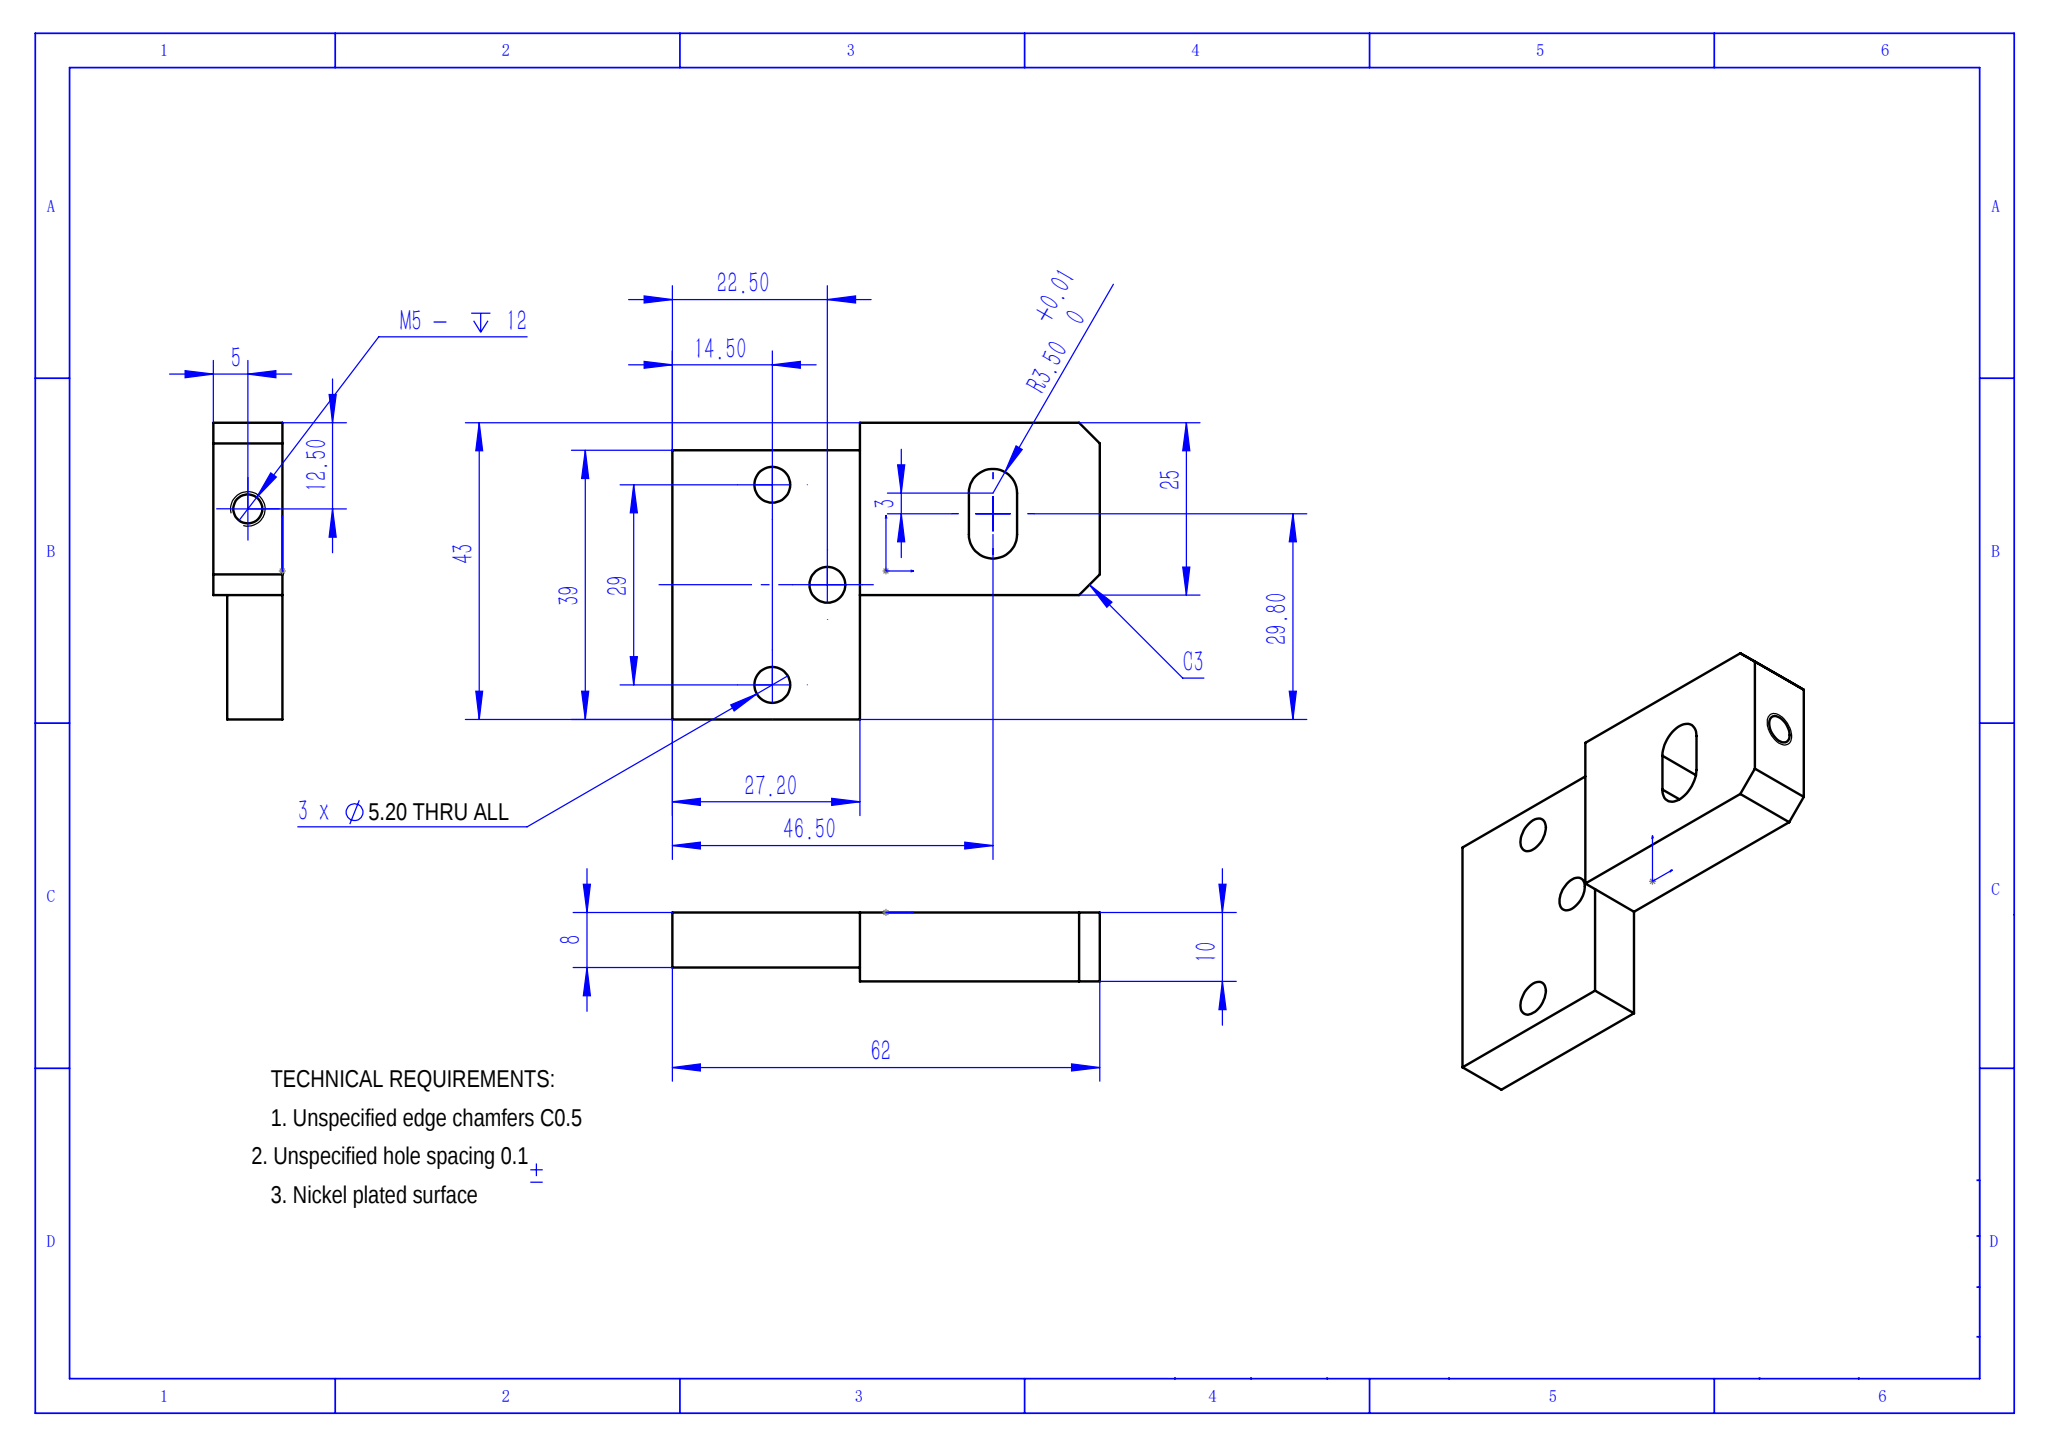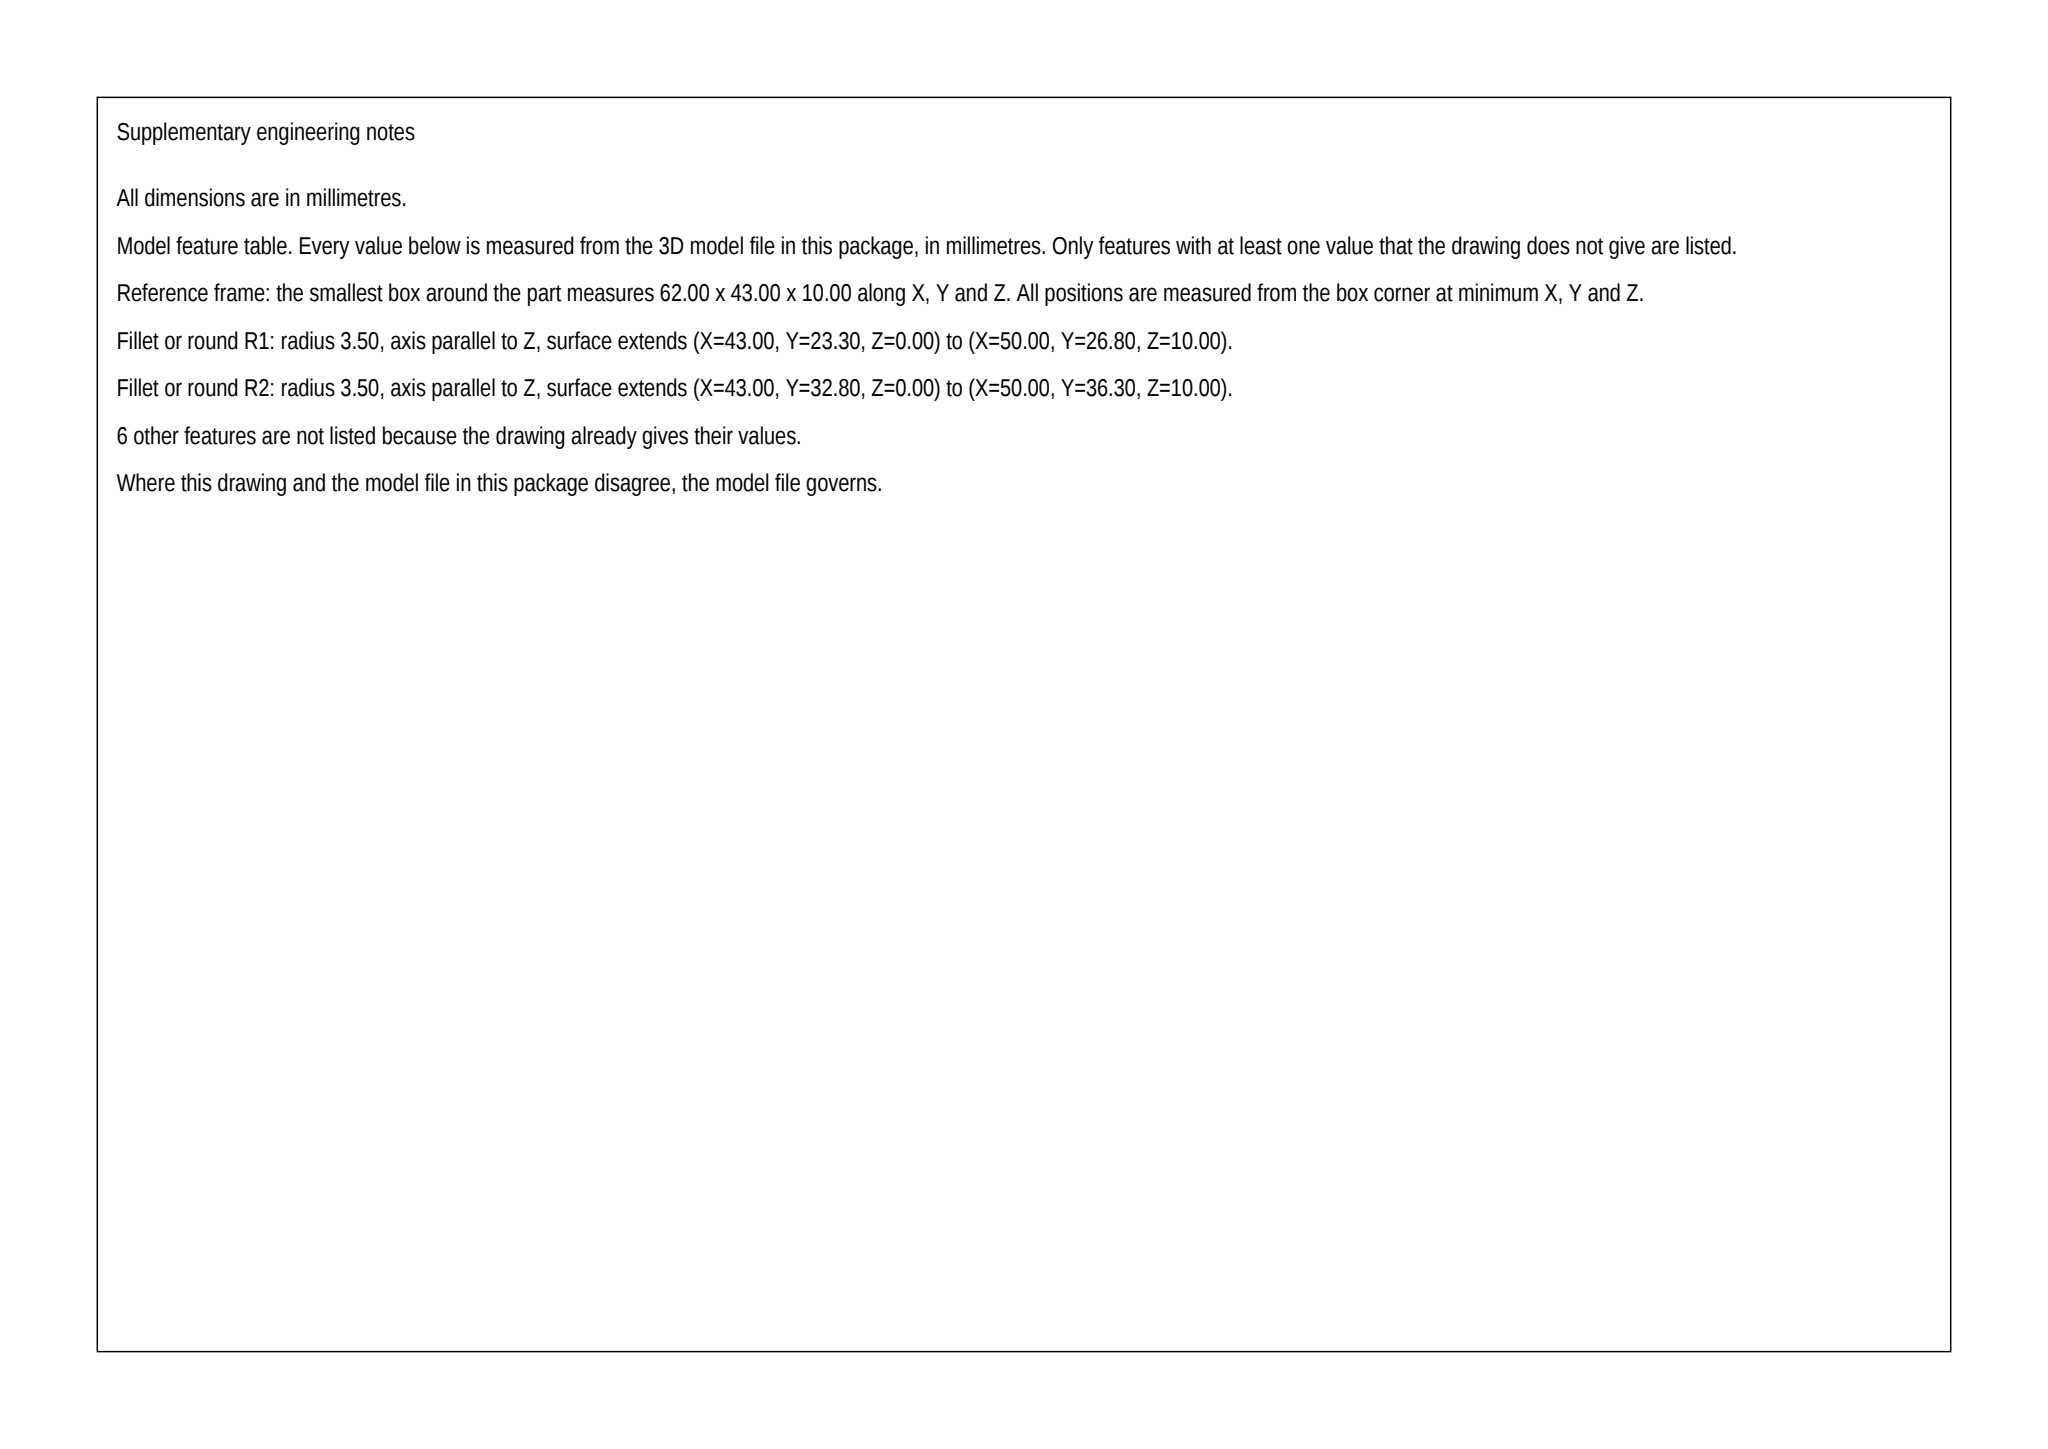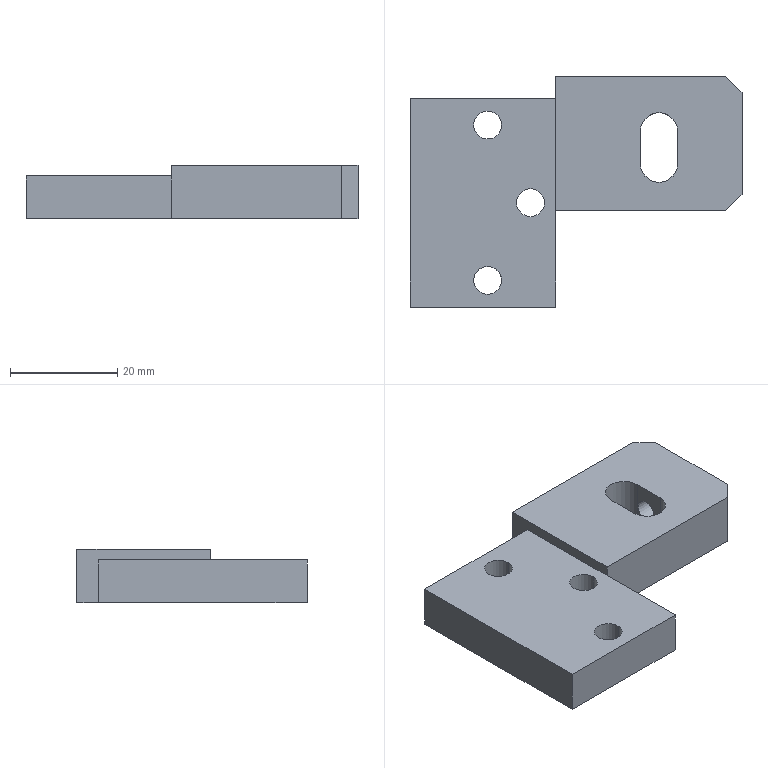Part | SolidWorks | mm | 1 solid | 25 faces | box 62 x 43 x 10 mm | volume 15616 mm3 | plane 15 | cylinder 10 | commonest cylinder face diameters 5.2 x6 4.2 x2 7 x2
build123d program:
from build123d import *

# Parameters (mm, degrees)
SKETCH1_W                  = 62
SKETCH1_H                  = 43
BOSS_EXTRUDE1_DEPTH        = 10
SKETCH2_W                  = 27.2
SKETCH2_H                  = 43
CUT_EXTRUDE1_DEPTH         = 2
SKETCH3_W                  = 27.2
SKETCH3_H                  = 4
CUT_EXTRUDE2_DEPTH         = 39.565
SKETCH7_W                  = 34.8
SKETCH7_H                  = 18
CUT_EXTRUDE3_DEPTH         = 40.029
F_5_2_5_2_DIAMETER_HOLE1_D = 5.2
CUT_EXTRUDE4_DEPTH         = 40.029
CHAMFER1_SIZE              = 3
M5_TAPPED_HOLE1_D          = 4.2
M5_TAPPED_HOLE1_DEPTH      = 14.4
M5_TAPPED_HOLE1_TIP        = 1.262


with BuildPart() as part:
    # Sketch1 → Boss-Extrude1 (new body)
    with BuildSketch(Plane.XY):
        Rectangle(SKETCH1_W, SKETCH1_H)
    extrude(amount=BOSS_EXTRUDE1_DEPTH)

    # Sketch2 → Cut-Extrude1 (cut)
    with BuildSketch(Plane.XY.offset(10)):
        with Locations((-17.4, 0)):
            Rectangle(SKETCH2_W, SKETCH2_H)
    extrude(amount=-CUT_EXTRUDE1_DEPTH, mode=Mode.SUBTRACT)

    # Sketch3 → Cut-Extrude2 (cut, through all)
    with BuildSketch(Plane.XY.offset(8)):
        with Locations((-17.4, 19.5)):
            Rectangle(SKETCH3_W, SKETCH3_H)
    extrude(amount=-CUT_EXTRUDE2_DEPTH, mode=Mode.SUBTRACT)

    # Sketch7 → Cut-Extrude3 (cut, through all)
    with BuildSketch(Plane.XY.offset(10)):
        with Locations((13.6, -12.5)):
            Rectangle(SKETCH7_W, SKETCH7_H)
    extrude(amount=-CUT_EXTRUDE3_DEPTH, mode=Mode.SUBTRACT)

    # 5.2 _5.2_ Diameter Hole1 (through all)
    with Locations(Plane(origin=(-16.5, 12.5, 0), x_dir=(-1, 0, 0), z_dir=(0, 0, -1))):
        with Locations((0, 0), (0, -29), (-8, -14.5)):
            Hole(F_5_2_5_2_DIAMETER_HOLE1_D / 2)

    # Sketch11 → Cut-Extrude4 (cut, through all)
    with BuildSketch(Plane.XY.offset(10)):
        with BuildLine():
            Line((12, 5.3), (12, 11.3))
            ThreePointArc((12, 11.3), (15.5, 14.8), (19, 11.3))
            Line((19, 11.3), (19, 5.3))
            ThreePointArc((19, 5.3), (15.5, 1.8), (12, 5.3))
        make_face()
    extrude(amount=-CUT_EXTRUDE4_DEPTH, mode=Mode.SUBTRACT)

    # Chamfer1
    chamfer1_edges = [part.edges().sort_by_distance(p)[0] for p in [
        (31, -3.5, 5),
        (31, 21.5, 5),
    ]]
    chamfer(chamfer1_edges, length=CHAMFER1_SIZE)

    # M5 Tapped Hole1
    with Locations(Plane(origin=(31, 9, 5), x_dir=(0, 1, 0), z_dir=(1, 0, 0))):
        with Locations((0, 0)):
            Hole(M5_TAPPED_HOLE1_D / 2, depth=M5_TAPPED_HOLE1_DEPTH)
            with Locations((0, 0, -(M5_TAPPED_HOLE1_DEPTH + M5_TAPPED_HOLE1_TIP / 2))):  # 118° drill point
                Cone(0, M5_TAPPED_HOLE1_D / 2, M5_TAPPED_HOLE1_TIP, mode=Mode.SUBTRACT)


solid = part.part
STEP:
#1=CARTESIAN_POINT('',(19.,9.,7.1));
#2=VERTEX_POINT('',#1);
#3=CARTESIAN_POINT('',(19.,9.,2.9));
#4=VERTEX_POINT('',#3);
#5=CARTESIAN_POINT('',(19.,9.,5.));
#6=DIRECTION('',(1.,0.,0.));
#7=DIRECTION('',(0.,0.,-1.));
#8=AXIS2_PLACEMENT_3D('',#5,#6,#7);
#9=CIRCLE('',#8,2.1);
#10=EDGE_CURVE('',#2,#4,#9,.T.);
#11=ORIENTED_EDGE('',*,*,#10,.F.);
#12=CARTESIAN_POINT('',(31.,9.,7.1));
#13=VERTEX_POINT('',#12);
#14=CARTESIAN_POINT('',(31.,9.,7.1));
#15=DIRECTION('',(1.,0.,0.));
#16=VECTOR('',#15,1000.);
#17=LINE('',#14,#16);
#18=EDGE_CURVE('',#2,#13,#17,.T.);
#19=ORIENTED_EDGE('',*,*,#18,.T.);
#20=CARTESIAN_POINT('',(31.,9.,2.9));
#21=VERTEX_POINT('',#20);
#22=CARTESIAN_POINT('',(31.,9.,5.));
#23=DIRECTION('',(1.,0.,0.));
#24=DIRECTION('',(0.,0.,-1.));
#25=AXIS2_PLACEMENT_3D('',#22,#23,#24);
#26=CIRCLE('',#25,2.1);
#27=EDGE_CURVE('',#13,#21,#26,.T.);
#28=ORIENTED_EDGE('',*,*,#27,.T.);
#29=CARTESIAN_POINT('',(31.,9.,2.9));
#30=DIRECTION('',(1.,0.,0.));
#31=VECTOR('',#30,1000.);
#32=LINE('',#29,#31);
#33=EDGE_CURVE('',#4,#21,#32,.T.);
#34=ORIENTED_EDGE('',*,*,#33,.F.);
#35=EDGE_LOOP('',(#11,#19,#28,#34));
#36=FACE_OUTER_BOUND('',#35,.T.);
#37=CARTESIAN_POINT('',(31.,9.,5.));
#38=DIRECTION('',(1.,0.,0.));
#39=DIRECTION('',(0.,0.,-1.));
#40=AXIS2_PLACEMENT_3D('',#37,#38,#39);
#41=CYLINDRICAL_SURFACE('',#40,2.1);
#42=ADVANCED_FACE('',(#36),#41,.F.);
#43=CARTESIAN_POINT('',(-19.1,12.5,8.));
#44=VERTEX_POINT('',#43);
#45=CARTESIAN_POINT('',(-13.9,12.5,8.));
#46=VERTEX_POINT('',#45);
#47=CARTESIAN_POINT('',(-16.5,12.5,8.));
#48=DIRECTION('',(0.,0.,1.));
#49=DIRECTION('',(1.,0.,0.));
#50=AXIS2_PLACEMENT_3D('',#47,#48,#49);
#51=CIRCLE('',#50,2.6);
#52=EDGE_CURVE('',#44,#46,#51,.T.);
#53=ORIENTED_EDGE('',*,*,#52,.T.);
#54=CARTESIAN_POINT('',(-13.9,12.5,0.));
#55=VERTEX_POINT('',#54);
#56=CARTESIAN_POINT('',(-13.9,12.5,0.));
#57=DIRECTION('',(0.,0.,-1.));
#58=VECTOR('',#57,1000.);
#59=LINE('',#56,#58);
#60=EDGE_CURVE('',#46,#55,#59,.T.);
#61=ORIENTED_EDGE('',*,*,#60,.T.);
#62=CARTESIAN_POINT('',(-19.1,12.5,0.));
#63=VERTEX_POINT('',#62);
#64=CARTESIAN_POINT('',(-16.5,12.5,0.));
#65=DIRECTION('',(0.,0.,-1.));
#66=DIRECTION('',(-1.,0.,0.));
#67=AXIS2_PLACEMENT_3D('',#64,#65,#66);
#68=CIRCLE('',#67,2.6);
#69=EDGE_CURVE('',#55,#63,#68,.T.);
#70=ORIENTED_EDGE('',*,*,#69,.T.);
#71=CARTESIAN_POINT('',(-19.1,12.5,0.));
#72=DIRECTION('',(0.,0.,-1.));
#73=VECTOR('',#72,1000.);
#74=LINE('',#71,#73);
#75=EDGE_CURVE('',#44,#63,#74,.T.);
#76=ORIENTED_EDGE('',*,*,#75,.F.);
#77=EDGE_LOOP('',(#53,#61,#70,#76));
#78=FACE_OUTER_BOUND('',#77,.T.);
#79=CARTESIAN_POINT('',(-16.5,12.5,0.));
#80=DIRECTION('',(0.,0.,-1.));
#81=DIRECTION('',(-1.,0.,0.));
#82=AXIS2_PLACEMENT_3D('',#79,#80,#81);
#83=CYLINDRICAL_SURFACE('',#82,2.6);
#84=ADVANCED_FACE('',(#78),#83,.F.);
#85=CARTESIAN_POINT('',(-19.1,-16.5,8.));
#86=VERTEX_POINT('',#85);
#87=CARTESIAN_POINT('',(-13.9,-16.5,8.));
#88=VERTEX_POINT('',#87);
#89=CARTESIAN_POINT('',(-16.5,-16.5,8.));
#90=DIRECTION('',(0.,0.,1.));
#91=DIRECTION('',(1.,0.,0.));
#92=AXIS2_PLACEMENT_3D('',#89,#90,#91);
#93=CIRCLE('',#92,2.6);
#94=EDGE_CURVE('',#86,#88,#93,.T.);
#95=ORIENTED_EDGE('',*,*,#94,.T.);
#96=CARTESIAN_POINT('',(-13.9,-16.5,0.));
#97=VERTEX_POINT('',#96);
#98=CARTESIAN_POINT('',(-13.9,-16.5,0.));
#99=DIRECTION('',(0.,0.,-1.));
#100=VECTOR('',#99,1000.);
#101=LINE('',#98,#100);
#102=EDGE_CURVE('',#88,#97,#101,.T.);
#103=ORIENTED_EDGE('',*,*,#102,.T.);
#104=CARTESIAN_POINT('',(-19.1,-16.5,0.));
#105=VERTEX_POINT('',#104);
#106=CARTESIAN_POINT('',(-16.5,-16.5,0.));
#107=DIRECTION('',(0.,0.,-1.));
#108=DIRECTION('',(-1.,0.,0.));
#109=AXIS2_PLACEMENT_3D('',#106,#107,#108);
#110=CIRCLE('',#109,2.6);
#111=EDGE_CURVE('',#97,#105,#110,.T.);
#112=ORIENTED_EDGE('',*,*,#111,.T.);
#113=CARTESIAN_POINT('',(-19.1,-16.5,0.));
#114=DIRECTION('',(0.,0.,-1.));
#115=VECTOR('',#114,1000.);
#116=LINE('',#113,#115);
#117=EDGE_CURVE('',#86,#105,#116,.T.);
#118=ORIENTED_EDGE('',*,*,#117,.F.);
#119=EDGE_LOOP('',(#95,#103,#112,#118));
#120=FACE_OUTER_BOUND('',#119,.T.);
#121=CARTESIAN_POINT('',(-16.5,-16.5,0.));
#122=DIRECTION('',(0.,0.,-1.));
#123=DIRECTION('',(-1.,0.,0.));
#124=AXIS2_PLACEMENT_3D('',#121,#122,#123);
#125=CYLINDRICAL_SURFACE('',#124,2.6);
#126=ADVANCED_FACE('',(#120),#125,.F.);
#127=CARTESIAN_POINT('',(-11.1,-2.,8.));
#128=VERTEX_POINT('',#127);
#129=CARTESIAN_POINT('',(-5.9,-2.,8.));
#130=VERTEX_POINT('',#129);
#131=CARTESIAN_POINT('',(-8.5,-2.,8.));
#132=DIRECTION('',(0.,0.,1.));
#133=DIRECTION('',(1.,0.,0.));
#134=AXIS2_PLACEMENT_3D('',#131,#132,#133);
#135=CIRCLE('',#134,2.6);
#136=EDGE_CURVE('',#128,#130,#135,.T.);
#137=ORIENTED_EDGE('',*,*,#136,.T.);
#138=CARTESIAN_POINT('',(-5.9,-2.,0.));
#139=VERTEX_POINT('',#138);
#140=CARTESIAN_POINT('',(-5.9,-2.,0.));
#141=DIRECTION('',(0.,0.,-1.));
#142=VECTOR('',#141,1000.);
#143=LINE('',#140,#142);
#144=EDGE_CURVE('',#130,#139,#143,.T.);
#145=ORIENTED_EDGE('',*,*,#144,.T.);
#146=CARTESIAN_POINT('',(-11.1,-2.,0.));
#147=VERTEX_POINT('',#146);
#148=CARTESIAN_POINT('',(-8.5,-2.,0.));
#149=DIRECTION('',(0.,0.,-1.));
#150=DIRECTION('',(-1.,0.,0.));
#151=AXIS2_PLACEMENT_3D('',#148,#149,#150);
#152=CIRCLE('',#151,2.6);
#153=EDGE_CURVE('',#139,#147,#152,.T.);
#154=ORIENTED_EDGE('',*,*,#153,.T.);
#155=CARTESIAN_POINT('',(-11.1,-2.,0.));
#156=DIRECTION('',(0.,0.,-1.));
#157=VECTOR('',#156,1000.);
#158=LINE('',#155,#157);
#159=EDGE_CURVE('',#128,#147,#158,.T.);
#160=ORIENTED_EDGE('',*,*,#159,.F.);
#161=EDGE_LOOP('',(#137,#145,#154,#160));
#162=FACE_OUTER_BOUND('',#161,.T.);
#163=CARTESIAN_POINT('',(-8.5,-2.,0.));
#164=DIRECTION('',(0.,0.,-1.));
#165=DIRECTION('',(-1.,0.,0.));
#166=AXIS2_PLACEMENT_3D('',#163,#164,#165);
#167=CYLINDRICAL_SURFACE('',#166,2.6);
#168=ADVANCED_FACE('',(#162),#167,.F.);
#169=CARTESIAN_POINT('',(-31.,17.5,8.));
#170=VERTEX_POINT('',#169);
#171=CARTESIAN_POINT('',(-31.,-21.5,8.));
#172=VERTEX_POINT('',#171);
#173=CARTESIAN_POINT('',(-31.,21.5,8.));
#174=DIRECTION('',(0.,-1.,0.));
#175=VECTOR('',#174,1000.);
#176=LINE('',#173,#175);
#177=EDGE_CURVE('',#170,#172,#176,.T.);
#178=ORIENTED_EDGE('',*,*,#177,.F.);
#179=CARTESIAN_POINT('',(-31.,17.5,0.));
#180=VERTEX_POINT('',#179);
#181=CARTESIAN_POINT('',(-31.,17.5,0.));
#182=DIRECTION('',(0.,0.,1.));
#183=VECTOR('',#182,1000.);
#184=LINE('',#181,#183);
#185=EDGE_CURVE('',#180,#170,#184,.T.);
#186=ORIENTED_EDGE('',*,*,#185,.F.);
#187=CARTESIAN_POINT('',(-31.,-21.5,0.));
#188=VERTEX_POINT('',#187);
#189=CARTESIAN_POINT('',(-31.,21.5,0.));
#190=DIRECTION('',(0.,-1.,0.));
#191=VECTOR('',#190,1000.);
#192=LINE('',#189,#191);
#193=EDGE_CURVE('',#180,#188,#192,.T.);
#194=ORIENTED_EDGE('',*,*,#193,.T.);
#195=CARTESIAN_POINT('',(-31.,-21.5,10.));
#196=DIRECTION('',(0.,0.,-1.));
#197=VECTOR('',#196,1000.);
#198=LINE('',#195,#197);
#199=EDGE_CURVE('',#172,#188,#198,.T.);
#200=ORIENTED_EDGE('',*,*,#199,.F.);
#201=EDGE_LOOP('',(#178,#186,#194,#200));
#202=FACE_OUTER_BOUND('',#201,.T.);
#203=CARTESIAN_POINT('',(-31.,21.5,10.));
#204=DIRECTION('',(1.,0.,0.));
#205=DIRECTION('',(-0.,1.,0.));
#206=AXIS2_PLACEMENT_3D('',#203,#204,#205);
#207=PLANE('',#206);
#208=ADVANCED_FACE('',(#202),#207,.F.);
#209=CARTESIAN_POINT('',(31.,9.,5.));
#210=DIRECTION('',(1.,0.,0.));
#211=DIRECTION('',(0.,0.,-1.));
#212=AXIS2_PLACEMENT_3D('',#209,#210,#211);
#213=CIRCLE('',#212,2.1);
#214=EDGE_CURVE('',#21,#13,#213,.T.);
#215=ORIENTED_EDGE('',*,*,#214,.F.);
#216=ORIENTED_EDGE('',*,*,#27,.F.);
#217=EDGE_LOOP('',(#215,#216));
#218=FACE_BOUND('',#217,.T.);
#219=CARTESIAN_POINT('',(31.,-0.5,10.));
#220=VERTEX_POINT('',#219);
#221=CARTESIAN_POINT('',(31.,18.5,10.));
#222=VERTEX_POINT('',#221);
#223=CARTESIAN_POINT('',(31.,21.5,10.));
#224=DIRECTION('',(-0.,1.,0.));
#225=VECTOR('',#224,1000.);
#226=LINE('',#223,#225);
#227=EDGE_CURVE('',#220,#222,#226,.T.);
#228=ORIENTED_EDGE('',*,*,#227,.F.);
#229=CARTESIAN_POINT('',(31.,-0.5,0.));
#230=VERTEX_POINT('',#229);
#231=CARTESIAN_POINT('',(31.,-0.5,10.));
#232=DIRECTION('',(0.,0.,-1.));
#233=VECTOR('',#232,1000.);
#234=LINE('',#231,#233);
#235=EDGE_CURVE('',#220,#230,#234,.T.);
#236=ORIENTED_EDGE('',*,*,#235,.T.);
#237=CARTESIAN_POINT('',(31.,18.5,0.));
#238=VERTEX_POINT('',#237);
#239=CARTESIAN_POINT('',(31.,21.5,0.));
#240=DIRECTION('',(-0.,1.,0.));
#241=VECTOR('',#240,1000.);
#242=LINE('',#239,#241);
#243=EDGE_CURVE('',#230,#238,#242,.T.);
#244=ORIENTED_EDGE('',*,*,#243,.T.);
#245=CARTESIAN_POINT('',(31.,18.5,10.));
#246=DIRECTION('',(0.,0.,1.));
#247=VECTOR('',#246,1000.);
#248=LINE('',#245,#247);
#249=EDGE_CURVE('',#238,#222,#248,.T.);
#250=ORIENTED_EDGE('',*,*,#249,.T.);
#251=EDGE_LOOP('',(#228,#236,#244,#250));
#252=FACE_OUTER_BOUND('',#251,.T.);
#253=CARTESIAN_POINT('',(31.,21.5,10.));
#254=DIRECTION('',(-1.,-0.,0.));
#255=DIRECTION('',(0.,-1.,0.));
#256=AXIS2_PLACEMENT_3D('',#253,#254,#255);
#257=PLANE('',#256);
#258=ADVANCED_FACE('',(#218,#252),#257,.F.);
#259=CARTESIAN_POINT('',(28.,21.5,10.));
#260=VERTEX_POINT('',#259);
#261=CARTESIAN_POINT('',(-3.8,21.5,10.));
#262=VERTEX_POINT('',#261);
#263=CARTESIAN_POINT('',(-31.,21.5,10.));
#264=DIRECTION('',(-1.,0.,0.));
#265=VECTOR('',#264,1000.);
#266=LINE('',#263,#265);
#267=EDGE_CURVE('',#260,#262,#266,.T.);
#268=ORIENTED_EDGE('',*,*,#267,.F.);
#269=CARTESIAN_POINT('',(28.,21.5,0.));
#270=VERTEX_POINT('',#269);
#271=CARTESIAN_POINT('',(28.,21.5,10.));
#272=DIRECTION('',(0.,0.,-1.));
#273=VECTOR('',#272,1000.);
#274=LINE('',#271,#273);
#275=EDGE_CURVE('',#260,#270,#274,.T.);
#276=ORIENTED_EDGE('',*,*,#275,.T.);
#277=CARTESIAN_POINT('',(-3.8,21.5,0.));
#278=VERTEX_POINT('',#277);
#279=CARTESIAN_POINT('',(-31.,21.5,0.));
#280=DIRECTION('',(-1.,0.,0.));
#281=VECTOR('',#280,1000.);
#282=LINE('',#279,#281);
#283=EDGE_CURVE('',#270,#278,#282,.T.);
#284=ORIENTED_EDGE('',*,*,#283,.T.);
#285=CARTESIAN_POINT('',(-3.8,21.5,8.));
#286=DIRECTION('',(0.,0.,1.));
#287=VECTOR('',#286,1000.);
#288=LINE('',#285,#287);
#289=EDGE_CURVE('',#278,#262,#288,.T.);
#290=ORIENTED_EDGE('',*,*,#289,.T.);
#291=EDGE_LOOP('',(#268,#276,#284,#290));
#292=FACE_OUTER_BOUND('',#291,.T.);
#293=CARTESIAN_POINT('',(-31.,21.5,10.));
#294=DIRECTION('',(0.,-1.,0.));
#295=DIRECTION('',(0.,0.,-1.));
#296=AXIS2_PLACEMENT_3D('',#293,#294,#295);
#297=PLANE('',#296);
#298=ADVANCED_FACE('',(#292),#297,.F.);
#299=CARTESIAN_POINT('',(-3.8,-21.5,0.));
#300=VERTEX_POINT('',#299);
#301=CARTESIAN_POINT('',(-31.,-21.5,0.));
#302=DIRECTION('',(1.,0.,0.));
#303=VECTOR('',#302,1000.);
#304=LINE('',#301,#303);
#305=EDGE_CURVE('',#188,#300,#304,.T.);
#306=ORIENTED_EDGE('',*,*,#305,.T.);
#307=CARTESIAN_POINT('',(-3.8,-21.5,8.));
#308=VERTEX_POINT('',#307);
#309=CARTESIAN_POINT('',(-3.8,-21.5,0.));
#310=DIRECTION('',(0.,0.,1.));
#311=VECTOR('',#310,1000.);
#312=LINE('',#309,#311);
#313=EDGE_CURVE('',#300,#308,#312,.T.);
#314=ORIENTED_EDGE('',*,*,#313,.T.);
#315=CARTESIAN_POINT('',(-31.,-21.5,8.));
#316=DIRECTION('',(1.,0.,0.));
#317=VECTOR('',#316,1000.);
#318=LINE('',#315,#317);
#319=EDGE_CURVE('',#172,#308,#318,.T.);
#320=ORIENTED_EDGE('',*,*,#319,.F.);
#321=ORIENTED_EDGE('',*,*,#199,.T.);
#322=EDGE_LOOP('',(#306,#314,#320,#321));
#323=FACE_OUTER_BOUND('',#322,.T.);
#324=CARTESIAN_POINT('',(-31.,-21.5,10.));
#325=DIRECTION('',(0.,1.,0.));
#326=DIRECTION('',(0.,0.,1.));
#327=AXIS2_PLACEMENT_3D('',#324,#325,#326);
#328=PLANE('',#327);
#329=ADVANCED_FACE('',(#323),#328,.F.);
#330=CARTESIAN_POINT('',(12.,5.3,10.));
#331=VERTEX_POINT('',#330);
#332=CARTESIAN_POINT('',(19.,5.3,10.));
#333=VERTEX_POINT('',#332);
#334=CARTESIAN_POINT('',(15.5,5.3,10.));
#335=DIRECTION('',(0.,0.,1.));
#336=DIRECTION('',(1.,0.,0.));
#337=AXIS2_PLACEMENT_3D('',#334,#335,#336);
#338=CIRCLE('',#337,3.5);
#339=EDGE_CURVE('',#331,#333,#338,.T.);
#340=ORIENTED_EDGE('',*,*,#339,.F.);
#341=CARTESIAN_POINT('',(12.,11.3,10.));
#342=VERTEX_POINT('',#341);
#343=CARTESIAN_POINT('',(12.,5.3,10.));
#344=DIRECTION('',(0.,-1.,0.));
#345=VECTOR('',#344,1000.);
#346=LINE('',#343,#345);
#347=EDGE_CURVE('',#342,#331,#346,.T.);
#348=ORIENTED_EDGE('',*,*,#347,.F.);
#349=CARTESIAN_POINT('',(19.,11.3,10.));
#350=VERTEX_POINT('',#349);
#351=CARTESIAN_POINT('',(15.5,11.3,10.));
#352=DIRECTION('',(0.,0.,1.));
#353=DIRECTION('',(1.,0.,0.));
#354=AXIS2_PLACEMENT_3D('',#351,#352,#353);
#355=CIRCLE('',#354,3.5);
#356=EDGE_CURVE('',#350,#342,#355,.T.);
#357=ORIENTED_EDGE('',*,*,#356,.F.);
#358=CARTESIAN_POINT('',(19.,5.3,10.));
#359=DIRECTION('',(0.,1.,0.));
#360=VECTOR('',#359,1000.);
#361=LINE('',#358,#360);
#362=EDGE_CURVE('',#333,#350,#361,.T.);
#363=ORIENTED_EDGE('',*,*,#362,.F.);
#364=EDGE_LOOP('',(#340,#348,#357,#363));
#365=FACE_BOUND('',#364,.T.);
#366=CARTESIAN_POINT('',(28.,-3.5,10.));
#367=VERTEX_POINT('',#366);
#368=CARTESIAN_POINT('',(-3.8,-3.5,10.));
#369=VERTEX_POINT('',#368);
#370=CARTESIAN_POINT('',(-3.8,-3.5,10.));
#371=DIRECTION('',(-1.,0.,0.));
#372=VECTOR('',#371,1000.);
#373=LINE('',#370,#372);
#374=EDGE_CURVE('',#367,#369,#373,.T.);
#375=ORIENTED_EDGE('',*,*,#374,.F.);
#376=CARTESIAN_POINT('',(15.75,-15.75,10.));
#377=DIRECTION('',(0.7071,0.7071,0.));
#378=VECTOR('',#377,1000.);
#379=LINE('',#376,#378);
#380=EDGE_CURVE('',#367,#220,#379,.T.);
#381=ORIENTED_EDGE('',*,*,#380,.T.);
#382=ORIENTED_EDGE('',*,*,#227,.T.);
#383=CARTESIAN_POINT('',(24.75,24.75,10.));
#384=DIRECTION('',(-0.7071,0.7071,0.));
#385=VECTOR('',#384,1000.);
#386=LINE('',#383,#385);
#387=EDGE_CURVE('',#222,#260,#386,.T.);
#388=ORIENTED_EDGE('',*,*,#387,.T.);
#389=ORIENTED_EDGE('',*,*,#267,.T.);
#390=CARTESIAN_POINT('',(-3.8,21.5,10.));
#391=DIRECTION('',(-0.,1.,0.));
#392=VECTOR('',#391,1000.);
#393=LINE('',#390,#392);
#394=EDGE_CURVE('',#369,#262,#393,.T.);
#395=ORIENTED_EDGE('',*,*,#394,.F.);
#396=EDGE_LOOP('',(#375,#381,#382,#388,#389,#395));
#397=FACE_OUTER_BOUND('',#396,.T.);
#398=CARTESIAN_POINT('',(0.,0.,10.));
#399=DIRECTION('',(0.,0.,1.));
#400=DIRECTION('',(1.,0.,0.));
#401=AXIS2_PLACEMENT_3D('',#398,#399,#400);
#402=PLANE('',#401);
#403=ADVANCED_FACE('',(#365,#397),#402,.T.);
#404=CARTESIAN_POINT('',(12.,11.3,0.));
#405=VERTEX_POINT('',#404);
#406=CARTESIAN_POINT('',(12.,5.3,0.));
#407=VERTEX_POINT('',#406);
#408=CARTESIAN_POINT('',(12.,5.3,0.));
#409=DIRECTION('',(0.,-1.,0.));
#410=VECTOR('',#409,1000.);
#411=LINE('',#408,#410);
#412=EDGE_CURVE('',#405,#407,#411,.T.);
#413=ORIENTED_EDGE('',*,*,#412,.T.);
#414=CARTESIAN_POINT('',(19.,5.3,0.));
#415=VERTEX_POINT('',#414);
#416=CARTESIAN_POINT('',(15.5,5.3,0.));
#417=DIRECTION('',(0.,0.,1.));
#418=DIRECTION('',(1.,0.,0.));
#419=AXIS2_PLACEMENT_3D('',#416,#417,#418);
#420=CIRCLE('',#419,3.5);
#421=EDGE_CURVE('',#407,#415,#420,.T.);
#422=ORIENTED_EDGE('',*,*,#421,.T.);
#423=CARTESIAN_POINT('',(19.,11.3,0.));
#424=VERTEX_POINT('',#423);
#425=CARTESIAN_POINT('',(19.,5.3,0.));
#426=DIRECTION('',(0.,1.,0.));
#427=VECTOR('',#426,1000.);
#428=LINE('',#425,#427);
#429=EDGE_CURVE('',#415,#424,#428,.T.);
#430=ORIENTED_EDGE('',*,*,#429,.T.);
#431=CARTESIAN_POINT('',(15.5,11.3,0.));
#432=DIRECTION('',(0.,0.,1.));
#433=DIRECTION('',(1.,0.,0.));
#434=AXIS2_PLACEMENT_3D('',#431,#432,#433);
#435=CIRCLE('',#434,3.5);
#436=EDGE_CURVE('',#424,#405,#435,.T.);
#437=ORIENTED_EDGE('',*,*,#436,.T.);
#438=EDGE_LOOP('',(#413,#422,#430,#437));
#439=FACE_BOUND('',#438,.T.);
#440=CARTESIAN_POINT('',(-16.5,12.5,0.));
#441=DIRECTION('',(0.,0.,-1.));
#442=DIRECTION('',(-1.,0.,0.));
#443=AXIS2_PLACEMENT_3D('',#440,#441,#442);
#444=CIRCLE('',#443,2.6);
#445=EDGE_CURVE('',#63,#55,#444,.T.);
#446=ORIENTED_EDGE('',*,*,#445,.F.);
#447=ORIENTED_EDGE('',*,*,#69,.F.);
#448=EDGE_LOOP('',(#446,#447));
#449=FACE_BOUND('',#448,.T.);
#450=CARTESIAN_POINT('',(-16.5,-16.5,0.));
#451=DIRECTION('',(0.,0.,-1.));
#452=DIRECTION('',(-1.,0.,0.));
#453=AXIS2_PLACEMENT_3D('',#450,#451,#452);
#454=CIRCLE('',#453,2.6);
#455=EDGE_CURVE('',#105,#97,#454,.T.);
#456=ORIENTED_EDGE('',*,*,#455,.F.);
#457=ORIENTED_EDGE('',*,*,#111,.F.);
#458=EDGE_LOOP('',(#456,#457));
#459=FACE_BOUND('',#458,.T.);
#460=CARTESIAN_POINT('',(-8.5,-2.,0.));
#461=DIRECTION('',(0.,0.,-1.));
#462=DIRECTION('',(-1.,0.,0.));
#463=AXIS2_PLACEMENT_3D('',#460,#461,#462);
#464=CIRCLE('',#463,2.6);
#465=EDGE_CURVE('',#147,#139,#464,.T.);
#466=ORIENTED_EDGE('',*,*,#465,.F.);
#467=ORIENTED_EDGE('',*,*,#153,.F.);
#468=EDGE_LOOP('',(#466,#467));
#469=FACE_BOUND('',#468,.T.);
#470=ORIENTED_EDGE('',*,*,#243,.F.);
#471=CARTESIAN_POINT('',(28.,-3.5,0.));
#472=VERTEX_POINT('',#471);
#473=CARTESIAN_POINT('',(28.,-3.5,0.));
#474=DIRECTION('',(-0.7071,-0.7071,0.));
#475=VECTOR('',#474,1000.);
#476=LINE('',#473,#475);
#477=EDGE_CURVE('',#230,#472,#476,.T.);
#478=ORIENTED_EDGE('',*,*,#477,.T.);
#479=CARTESIAN_POINT('',(-3.8,-3.5,0.));
#480=VERTEX_POINT('',#479);
#481=CARTESIAN_POINT('',(-3.8,-3.5,0.));
#482=DIRECTION('',(-1.,0.,0.));
#483=VECTOR('',#482,1000.);
#484=LINE('',#481,#483);
#485=EDGE_CURVE('',#472,#480,#484,.T.);
#486=ORIENTED_EDGE('',*,*,#485,.T.);
#487=CARTESIAN_POINT('',(-3.8,-3.5,0.));
#488=DIRECTION('',(0.,-1.,0.));
#489=VECTOR('',#488,1000.);
#490=LINE('',#487,#489);
#491=EDGE_CURVE('',#480,#300,#490,.T.);
#492=ORIENTED_EDGE('',*,*,#491,.T.);
#493=ORIENTED_EDGE('',*,*,#305,.F.);
#494=ORIENTED_EDGE('',*,*,#193,.F.);
#495=CARTESIAN_POINT('',(-3.8,17.5,0.));
#496=VERTEX_POINT('',#495);
#497=CARTESIAN_POINT('',(-31.,17.5,0.));
#498=DIRECTION('',(1.,-0.,0.));
#499=VECTOR('',#498,1000.);
#500=LINE('',#497,#499);
#501=EDGE_CURVE('',#180,#496,#500,.T.);
#502=ORIENTED_EDGE('',*,*,#501,.T.);
#503=CARTESIAN_POINT('',(-3.8,21.5,0.));
#504=DIRECTION('',(0.,1.,0.));
#505=VECTOR('',#504,1000.);
#506=LINE('',#503,#505);
#507=EDGE_CURVE('',#496,#278,#506,.T.);
#508=ORIENTED_EDGE('',*,*,#507,.T.);
#509=ORIENTED_EDGE('',*,*,#283,.F.);
#510=CARTESIAN_POINT('',(28.,21.5,0.));
#511=DIRECTION('',(0.7071,-0.7071,0.));
#512=VECTOR('',#511,1000.);
#513=LINE('',#510,#512);
#514=EDGE_CURVE('',#270,#238,#513,.T.);
#515=ORIENTED_EDGE('',*,*,#514,.T.);
#516=EDGE_LOOP('',(#470,#478,#486,#492,#493,#494,#502,#508,#509,#515));
#517=FACE_OUTER_BOUND('',#516,.T.);
#518=CARTESIAN_POINT('',(0.,0.,0.));
#519=DIRECTION('',(0.,0.,1.));
#520=DIRECTION('',(1.,0.,0.));
#521=AXIS2_PLACEMENT_3D('',#518,#519,#520);
#522=PLANE('',#521);
#523=ADVANCED_FACE('',(#439,#449,#459,#469,#517),#522,.F.);
#524=CARTESIAN_POINT('',(-3.8,-3.5,8.));
#525=VERTEX_POINT('',#524);
#526=CARTESIAN_POINT('',(-3.8,17.5,8.));
#527=VERTEX_POINT('',#526);
#528=CARTESIAN_POINT('',(-3.8,21.5,8.));
#529=DIRECTION('',(-0.,1.,0.));
#530=VECTOR('',#529,1000.);
#531=LINE('',#528,#530);
#532=EDGE_CURVE('',#525,#527,#531,.T.);
#533=ORIENTED_EDGE('',*,*,#532,.F.);
#534=CARTESIAN_POINT('',(-3.8,-3.5,0.));
#535=DIRECTION('',(0.,0.,1.));
#536=VECTOR('',#535,1000.);
#537=LINE('',#534,#536);
#538=EDGE_CURVE('',#525,#369,#537,.T.);
#539=ORIENTED_EDGE('',*,*,#538,.T.);
#540=ORIENTED_EDGE('',*,*,#394,.T.);
#541=ORIENTED_EDGE('',*,*,#289,.F.);
#542=ORIENTED_EDGE('',*,*,#507,.F.);
#543=CARTESIAN_POINT('',(-3.8,17.5,0.));
#544=DIRECTION('',(0.,0.,1.));
#545=VECTOR('',#544,1000.);
#546=LINE('',#543,#545);
#547=EDGE_CURVE('',#496,#527,#546,.T.);
#548=ORIENTED_EDGE('',*,*,#547,.T.);
#549=EDGE_LOOP('',(#533,#539,#540,#541,#542,#548));
#550=FACE_OUTER_BOUND('',#549,.T.);
#551=CARTESIAN_POINT('',(-3.8,21.5,8.));
#552=DIRECTION('',(1.,0.,0.));
#553=DIRECTION('',(-0.,1.,0.));
#554=AXIS2_PLACEMENT_3D('',#551,#552,#553);
#555=PLANE('',#554);
#556=ADVANCED_FACE('',(#550),#555,.F.);
#557=ORIENTED_EDGE('',*,*,#52,.F.);
#558=CARTESIAN_POINT('',(-16.5,12.5,8.));
#559=DIRECTION('',(0.,0.,1.));
#560=DIRECTION('',(1.,0.,0.));
#561=AXIS2_PLACEMENT_3D('',#558,#559,#560);
#562=CIRCLE('',#561,2.6);
#563=EDGE_CURVE('',#46,#44,#562,.T.);
#564=ORIENTED_EDGE('',*,*,#563,.F.);
#565=EDGE_LOOP('',(#557,#564));
#566=FACE_BOUND('',#565,.T.);
#567=ORIENTED_EDGE('',*,*,#94,.F.);
#568=CARTESIAN_POINT('',(-16.5,-16.5,8.));
#569=DIRECTION('',(0.,0.,1.));
#570=DIRECTION('',(1.,0.,0.));
#571=AXIS2_PLACEMENT_3D('',#568,#569,#570);
#572=CIRCLE('',#571,2.6);
#573=EDGE_CURVE('',#88,#86,#572,.T.);
#574=ORIENTED_EDGE('',*,*,#573,.F.);
#575=EDGE_LOOP('',(#567,#574));
#576=FACE_BOUND('',#575,.T.);
#577=ORIENTED_EDGE('',*,*,#136,.F.);
#578=CARTESIAN_POINT('',(-8.5,-2.,8.));
#579=DIRECTION('',(0.,0.,1.));
#580=DIRECTION('',(1.,0.,0.));
#581=AXIS2_PLACEMENT_3D('',#578,#579,#580);
#582=CIRCLE('',#581,2.6);
#583=EDGE_CURVE('',#130,#128,#582,.T.);
#584=ORIENTED_EDGE('',*,*,#583,.F.);
#585=EDGE_LOOP('',(#577,#584));
#586=FACE_BOUND('',#585,.T.);
#587=CARTESIAN_POINT('',(-31.,17.5,8.));
#588=DIRECTION('',(1.,-0.,0.));
#589=VECTOR('',#588,1000.);
#590=LINE('',#587,#589);
#591=EDGE_CURVE('',#170,#527,#590,.T.);
#592=ORIENTED_EDGE('',*,*,#591,.F.);
#593=ORIENTED_EDGE('',*,*,#177,.T.);
#594=ORIENTED_EDGE('',*,*,#319,.T.);
#595=CARTESIAN_POINT('',(-3.8,21.5,8.));
#596=DIRECTION('',(-0.,1.,0.));
#597=VECTOR('',#596,1000.);
#598=LINE('',#595,#597);
#599=EDGE_CURVE('',#308,#525,#598,.T.);
#600=ORIENTED_EDGE('',*,*,#599,.T.);
#601=ORIENTED_EDGE('',*,*,#532,.T.);
#602=EDGE_LOOP('',(#592,#593,#594,#600,#601));
#603=FACE_OUTER_BOUND('',#602,.T.);
#604=CARTESIAN_POINT('',(0.,0.,8.));
#605=DIRECTION('',(0.,0.,1.));
#606=DIRECTION('',(1.,0.,0.));
#607=AXIS2_PLACEMENT_3D('',#604,#605,#606);
#608=PLANE('',#607);
#609=ADVANCED_FACE('',(#566,#576,#586,#603),#608,.T.);
#610=ORIENTED_EDGE('',*,*,#591,.T.);
#611=ORIENTED_EDGE('',*,*,#547,.F.);
#612=ORIENTED_EDGE('',*,*,#501,.F.);
#613=ORIENTED_EDGE('',*,*,#185,.T.);
#614=EDGE_LOOP('',(#610,#611,#612,#613));
#615=FACE_OUTER_BOUND('',#614,.T.);
#616=CARTESIAN_POINT('',(-31.,17.5,0.));
#617=DIRECTION('',(-0.,-1.,0.));
#618=DIRECTION('',(1.,-0.,0.));
#619=AXIS2_PLACEMENT_3D('',#616,#617,#618);
#620=PLANE('',#619);
#621=ADVANCED_FACE('',(#615),#620,.F.);
#622=ORIENTED_EDGE('',*,*,#599,.F.);
#623=ORIENTED_EDGE('',*,*,#313,.F.);
#624=ORIENTED_EDGE('',*,*,#491,.F.);
#625=CARTESIAN_POINT('',(-3.8,-3.5,0.));
#626=DIRECTION('',(0.,0.,1.));
#627=VECTOR('',#626,1000.);
#628=LINE('',#625,#627);
#629=EDGE_CURVE('',#480,#525,#628,.T.);
#630=ORIENTED_EDGE('',*,*,#629,.T.);
#631=EDGE_LOOP('',(#622,#623,#624,#630));
#632=FACE_OUTER_BOUND('',#631,.T.);
#633=CARTESIAN_POINT('',(-3.8,-3.5,0.));
#634=DIRECTION('',(-1.,-0.,0.));
#635=DIRECTION('',(0.,-1.,0.));
#636=AXIS2_PLACEMENT_3D('',#633,#634,#635);
#637=PLANE('',#636);
#638=ADVANCED_FACE('',(#632),#637,.F.);
#639=ORIENTED_EDGE('',*,*,#485,.F.);
#640=CARTESIAN_POINT('',(28.,-3.5,0.));
#641=DIRECTION('',(0.,0.,1.));
#642=VECTOR('',#641,1000.);
#643=LINE('',#640,#642);
#644=EDGE_CURVE('',#472,#367,#643,.T.);
#645=ORIENTED_EDGE('',*,*,#644,.T.);
#646=ORIENTED_EDGE('',*,*,#374,.T.);
#647=ORIENTED_EDGE('',*,*,#538,.F.);
#648=ORIENTED_EDGE('',*,*,#629,.F.);
#649=EDGE_LOOP('',(#639,#645,#646,#647,#648));
#650=FACE_OUTER_BOUND('',#649,.T.);
#651=CARTESIAN_POINT('',(-3.8,-3.5,0.));
#652=DIRECTION('',(0.,1.,0.));
#653=DIRECTION('',(0.,0.,1.));
#654=AXIS2_PLACEMENT_3D('',#651,#652,#653);
#655=PLANE('',#654);
#656=ADVANCED_FACE('',(#650),#655,.F.);
#657=ORIENTED_EDGE('',*,*,#144,.F.);
#658=ORIENTED_EDGE('',*,*,#583,.T.);
#659=ORIENTED_EDGE('',*,*,#159,.T.);
#660=ORIENTED_EDGE('',*,*,#465,.T.);
#661=EDGE_LOOP('',(#657,#658,#659,#660));
#662=FACE_OUTER_BOUND('',#661,.T.);
#663=CARTESIAN_POINT('',(-8.5,-2.,0.));
#664=DIRECTION('',(0.,0.,-1.));
#665=DIRECTION('',(-1.,0.,0.));
#666=AXIS2_PLACEMENT_3D('',#663,#664,#665);
#667=CYLINDRICAL_SURFACE('',#666,2.6);
#668=ADVANCED_FACE('',(#662),#667,.F.);
#669=ORIENTED_EDGE('',*,*,#102,.F.);
#670=ORIENTED_EDGE('',*,*,#573,.T.);
#671=ORIENTED_EDGE('',*,*,#117,.T.);
#672=ORIENTED_EDGE('',*,*,#455,.T.);
#673=EDGE_LOOP('',(#669,#670,#671,#672));
#674=FACE_OUTER_BOUND('',#673,.T.);
#675=CARTESIAN_POINT('',(-16.5,-16.5,0.));
#676=DIRECTION('',(0.,0.,-1.));
#677=DIRECTION('',(-1.,0.,0.));
#678=AXIS2_PLACEMENT_3D('',#675,#676,#677);
#679=CYLINDRICAL_SURFACE('',#678,2.6);
#680=ADVANCED_FACE('',(#674),#679,.F.);
#681=ORIENTED_EDGE('',*,*,#60,.F.);
#682=ORIENTED_EDGE('',*,*,#563,.T.);
#683=ORIENTED_EDGE('',*,*,#75,.T.);
#684=ORIENTED_EDGE('',*,*,#445,.T.);
#685=EDGE_LOOP('',(#681,#682,#683,#684));
#686=FACE_OUTER_BOUND('',#685,.T.);
#687=CARTESIAN_POINT('',(-16.5,12.5,0.));
#688=DIRECTION('',(0.,0.,-1.));
#689=DIRECTION('',(-1.,0.,0.));
#690=AXIS2_PLACEMENT_3D('',#687,#688,#689);
#691=CYLINDRICAL_SURFACE('',#690,2.6);
#692=ADVANCED_FACE('',(#686),#691,.F.);
#693=ORIENTED_EDGE('',*,*,#339,.T.);
#694=CARTESIAN_POINT('',(19.,5.3,0.));
#695=DIRECTION('',(0.,0.,1.));
#696=VECTOR('',#695,1000.);
#697=LINE('',#694,#696);
#698=EDGE_CURVE('',#415,#333,#697,.T.);
#699=ORIENTED_EDGE('',*,*,#698,.F.);
#700=ORIENTED_EDGE('',*,*,#421,.F.);
#701=CARTESIAN_POINT('',(12.,5.3,0.));
#702=DIRECTION('',(0.,0.,1.));
#703=VECTOR('',#702,1000.);
#704=LINE('',#701,#703);
#705=EDGE_CURVE('',#407,#331,#704,.T.);
#706=ORIENTED_EDGE('',*,*,#705,.T.);
#707=EDGE_LOOP('',(#693,#699,#700,#706));
#708=FACE_OUTER_BOUND('',#707,.T.);
#709=CARTESIAN_POINT('',(15.5,5.3,0.));
#710=DIRECTION('',(0.,0.,1.));
#711=DIRECTION('',(1.,0.,0.));
#712=AXIS2_PLACEMENT_3D('',#709,#710,#711);
#713=CYLINDRICAL_SURFACE('',#712,3.5);
#714=ADVANCED_FACE('',(#708),#713,.F.);
#715=ORIENTED_EDGE('',*,*,#347,.T.);
#716=ORIENTED_EDGE('',*,*,#705,.F.);
#717=ORIENTED_EDGE('',*,*,#412,.F.);
#718=CARTESIAN_POINT('',(12.,11.3,0.));
#719=DIRECTION('',(0.,0.,1.));
#720=VECTOR('',#719,1000.);
#721=LINE('',#718,#720);
#722=EDGE_CURVE('',#405,#342,#721,.T.);
#723=ORIENTED_EDGE('',*,*,#722,.T.);
#724=EDGE_LOOP('',(#715,#716,#717,#723));
#725=FACE_OUTER_BOUND('',#724,.T.);
#726=CARTESIAN_POINT('',(12.,5.3,0.));
#727=DIRECTION('',(-1.,0.,0.));
#728=DIRECTION('',(0.,0.,1.));
#729=AXIS2_PLACEMENT_3D('',#726,#727,#728);
#730=PLANE('',#729);
#731=ADVANCED_FACE('',(#725),#730,.F.);
#732=ORIENTED_EDGE('',*,*,#356,.T.);
#733=ORIENTED_EDGE('',*,*,#722,.F.);
#734=ORIENTED_EDGE('',*,*,#436,.F.);
#735=CARTESIAN_POINT('',(19.,11.3,0.));
#736=DIRECTION('',(0.,0.,1.));
#737=VECTOR('',#736,1000.);
#738=LINE('',#735,#737);
#739=EDGE_CURVE('',#424,#350,#738,.T.);
#740=ORIENTED_EDGE('',*,*,#739,.T.);
#741=EDGE_LOOP('',(#732,#733,#734,#740));
#742=FACE_OUTER_BOUND('',#741,.T.);
#743=CARTESIAN_POINT('',(15.5,11.3,0.));
#744=DIRECTION('',(0.,0.,1.));
#745=DIRECTION('',(1.,0.,0.));
#746=AXIS2_PLACEMENT_3D('',#743,#744,#745);
#747=CYLINDRICAL_SURFACE('',#746,3.5);
#748=ADVANCED_FACE('',(#742),#747,.F.);
#749=CARTESIAN_POINT('',(19.,9.,5.));
#750=DIRECTION('',(1.,0.,0.));
#751=DIRECTION('',(0.,0.,-1.));
#752=AXIS2_PLACEMENT_3D('',#749,#750,#751);
#753=CIRCLE('',#752,2.1);
#754=EDGE_CURVE('',#4,#2,#753,.T.);
#755=ORIENTED_EDGE('',*,*,#754,.T.);
#756=ORIENTED_EDGE('',*,*,#10,.T.);
#757=EDGE_LOOP('',(#755,#756));
#758=FACE_BOUND('',#757,.T.);
#759=ORIENTED_EDGE('',*,*,#362,.T.);
#760=ORIENTED_EDGE('',*,*,#739,.F.);
#761=ORIENTED_EDGE('',*,*,#429,.F.);
#762=ORIENTED_EDGE('',*,*,#698,.T.);
#763=EDGE_LOOP('',(#759,#760,#761,#762));
#764=FACE_OUTER_BOUND('',#763,.T.);
#765=CARTESIAN_POINT('',(19.,5.3,0.));
#766=DIRECTION('',(1.,0.,0.));
#767=DIRECTION('',(0.,0.,-1.));
#768=AXIS2_PLACEMENT_3D('',#765,#766,#767);
#769=PLANE('',#768);
#770=ADVANCED_FACE('',(#758,#764),#769,.F.);
#771=ORIENTED_EDGE('',*,*,#477,.F.);
#772=ORIENTED_EDGE('',*,*,#235,.F.);
#773=ORIENTED_EDGE('',*,*,#380,.F.);
#774=ORIENTED_EDGE('',*,*,#644,.F.);
#775=EDGE_LOOP('',(#771,#772,#773,#774));
#776=FACE_OUTER_BOUND('',#775,.T.);
#777=CARTESIAN_POINT('',(28.,-3.5,0.));
#778=DIRECTION('',(-0.7071,0.7071,0.));
#779=DIRECTION('',(0.,0.,1.));
#780=AXIS2_PLACEMENT_3D('',#777,#778,#779);
#781=PLANE('',#780);
#782=ADVANCED_FACE('',(#776),#781,.F.);
#783=ORIENTED_EDGE('',*,*,#387,.F.);
#784=ORIENTED_EDGE('',*,*,#249,.F.);
#785=ORIENTED_EDGE('',*,*,#514,.F.);
#786=ORIENTED_EDGE('',*,*,#275,.F.);
#787=EDGE_LOOP('',(#783,#784,#785,#786));
#788=FACE_OUTER_BOUND('',#787,.T.);
#789=CARTESIAN_POINT('',(28.,21.5,10.));
#790=DIRECTION('',(-0.7071,-0.7071,0.));
#791=DIRECTION('',(0.,0.,-1.));
#792=AXIS2_PLACEMENT_3D('',#789,#790,#791);
#793=PLANE('',#792);
#794=ADVANCED_FACE('',(#788),#793,.F.);
#795=ORIENTED_EDGE('',*,*,#18,.F.);
#796=ORIENTED_EDGE('',*,*,#754,.F.);
#797=ORIENTED_EDGE('',*,*,#33,.T.);
#798=ORIENTED_EDGE('',*,*,#214,.T.);
#799=EDGE_LOOP('',(#795,#796,#797,#798));
#800=FACE_OUTER_BOUND('',#799,.T.);
#801=CARTESIAN_POINT('',(31.,9.,5.));
#802=DIRECTION('',(1.,0.,0.));
#803=DIRECTION('',(0.,0.,-1.));
#804=AXIS2_PLACEMENT_3D('',#801,#802,#803);
#805=CYLINDRICAL_SURFACE('',#804,2.1);
#806=ADVANCED_FACE('',(#800),#805,.F.);
#807=CLOSED_SHELL('',(#42,#84,#126,#168,#208,#258,#298,#329,#403,#523,#556,#609,#621,#638,#656,#668,#680,#692,#714,#731,#748,#770,#782,#794,#806));
#808=MANIFOLD_SOLID_BREP('',#807);
#809=CARTESIAN_POINT('',(0.,0.,0.));
#810=DIRECTION('',(0.,0.,1.));
#811=DIRECTION('',(1.,0.,0.));
#812=AXIS2_PLACEMENT_3D('',#809,#810,#811);
#813=(LENGTH_UNIT()NAMED_UNIT(*)SI_UNIT(.MILLI.,.METRE.));
#814=UNCERTAINTY_MEASURE_WITH_UNIT(LENGTH_MEASURE(0.00001),#813,'','');
#815=(NAMED_UNIT(*)PLANE_ANGLE_UNIT()SI_UNIT($,.RADIAN.));
#816=(NAMED_UNIT(*)SI_UNIT($,.STERADIAN.)SOLID_ANGLE_UNIT());
#817=(GEOMETRIC_REPRESENTATION_CONTEXT(3)GLOBAL_UNCERTAINTY_ASSIGNED_CONTEXT((#814))GLOBAL_UNIT_ASSIGNED_CONTEXT((#813,#815,#816))REPRESENTATION_CONTEXT('',''));
#818=ADVANCED_BREP_SHAPE_REPRESENTATION('',(#808,#812),#817);